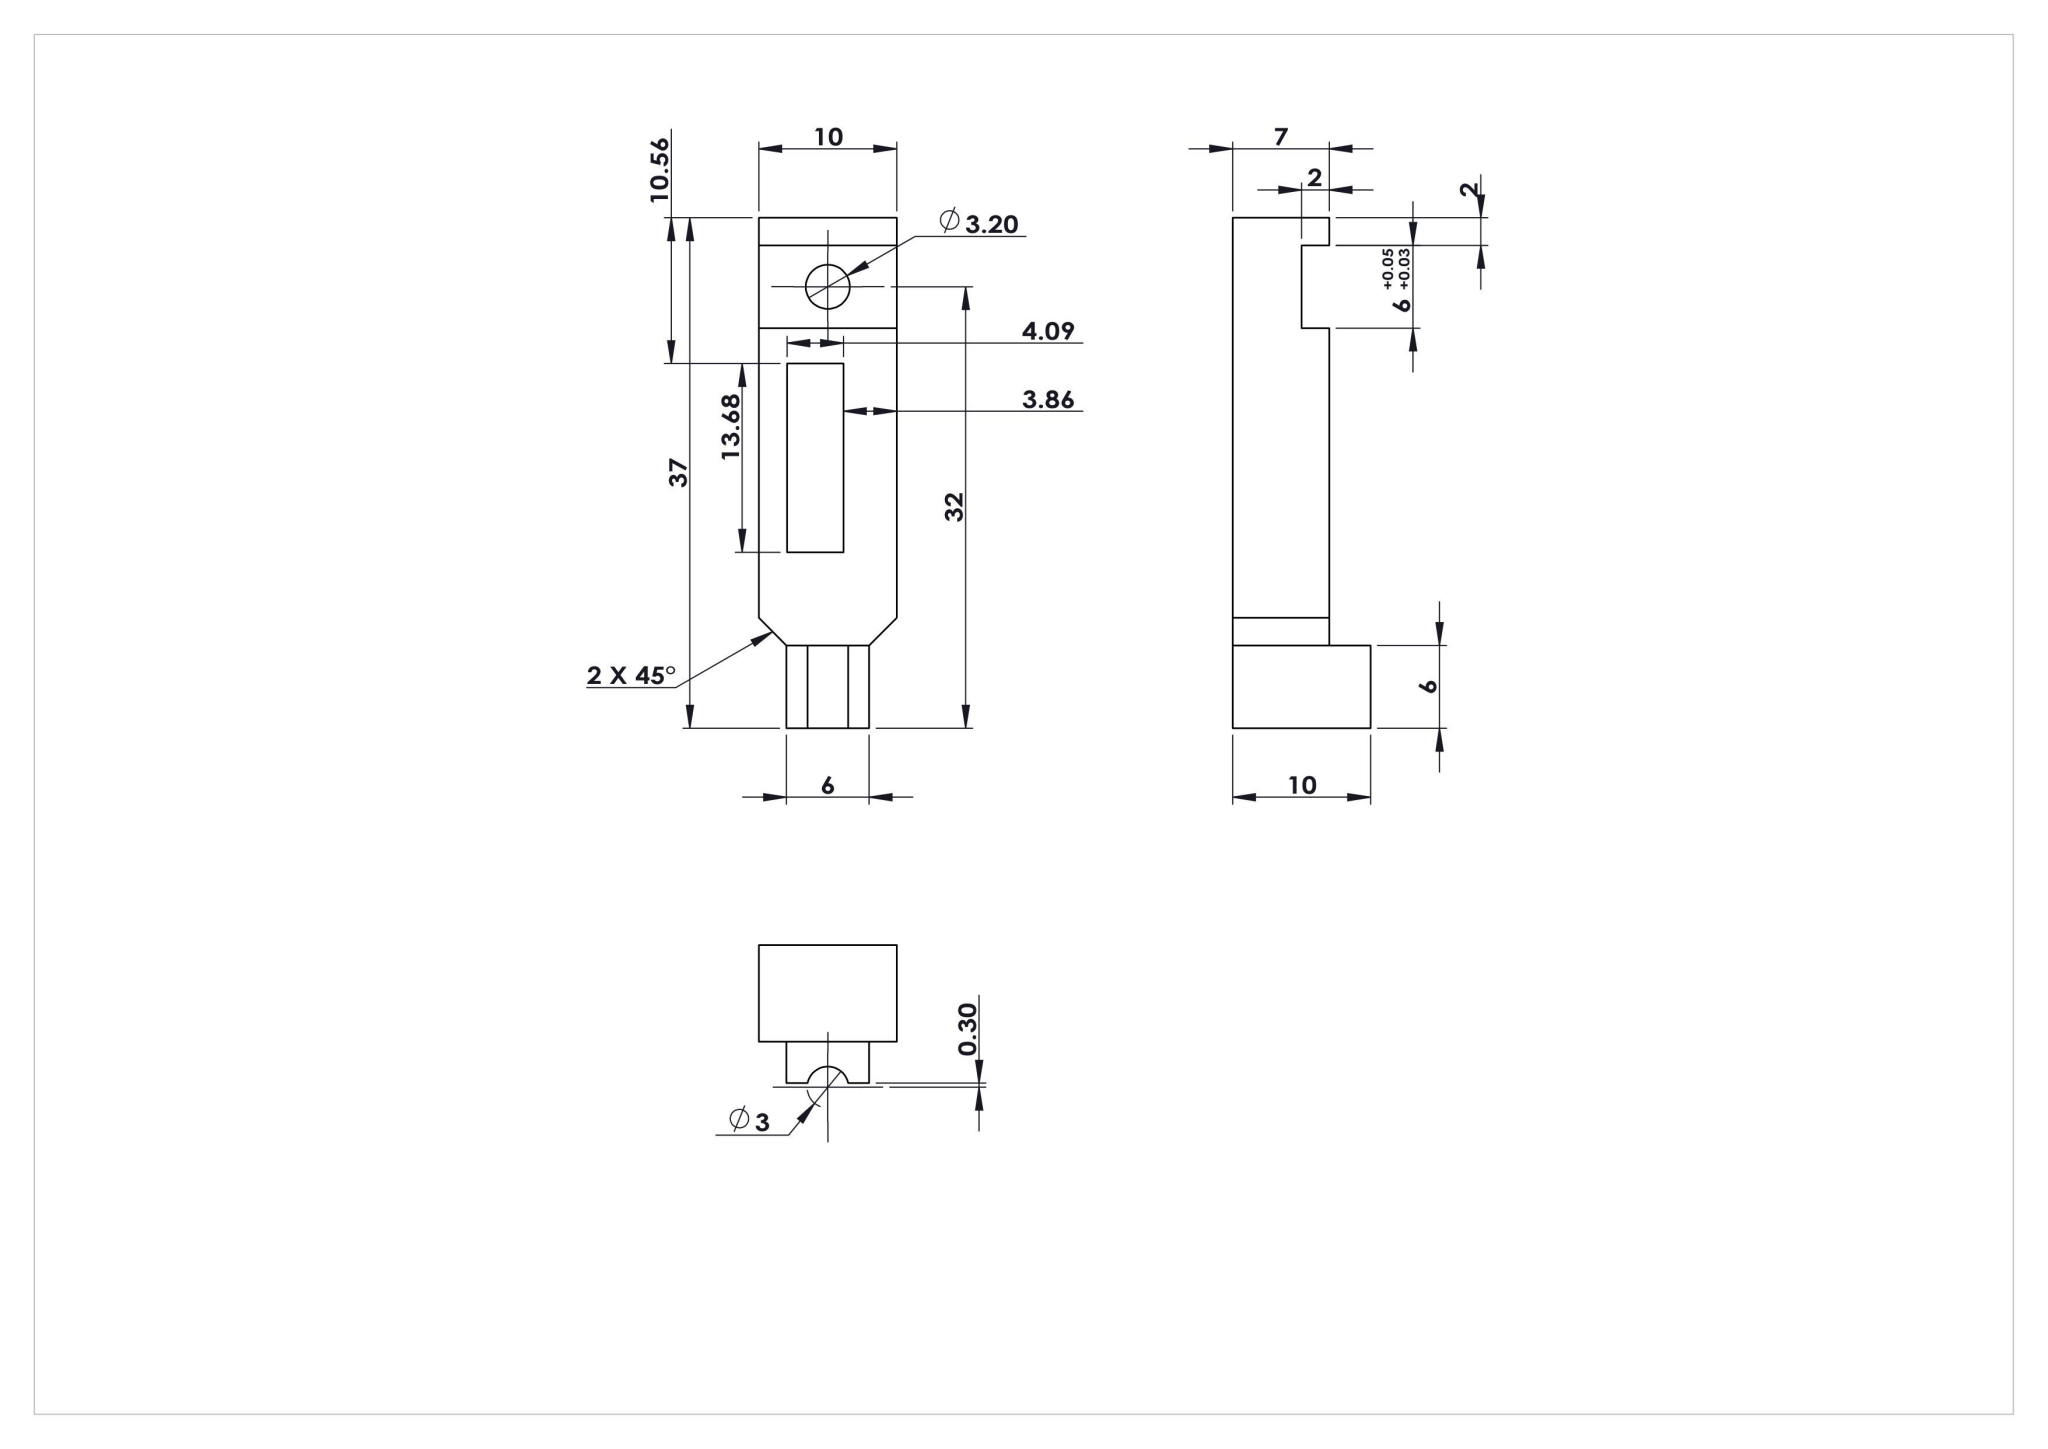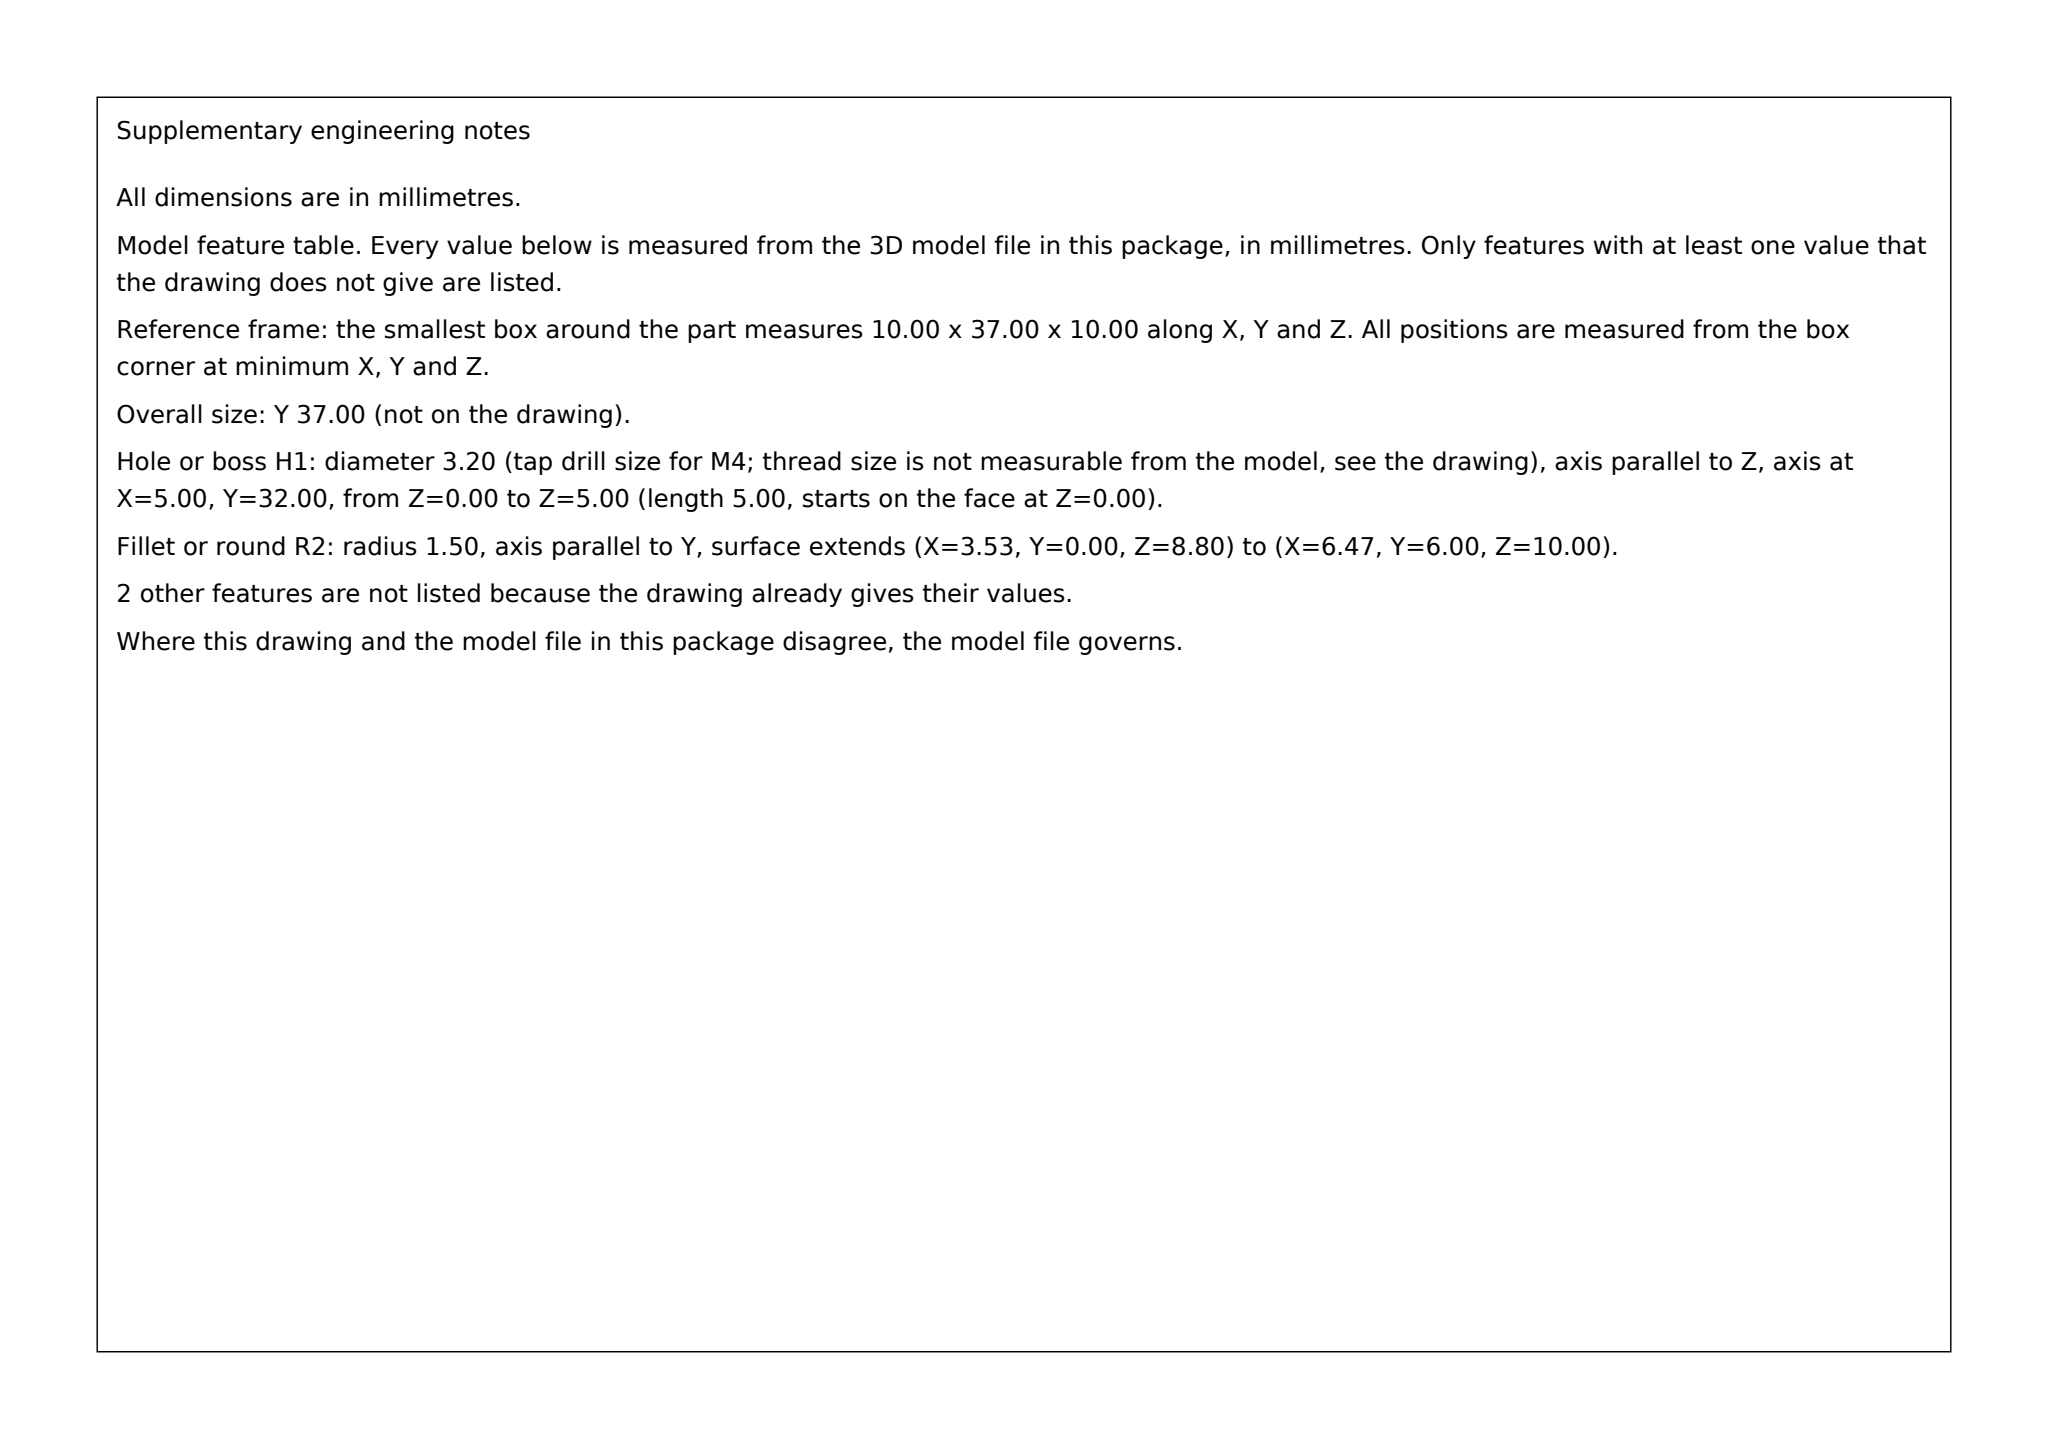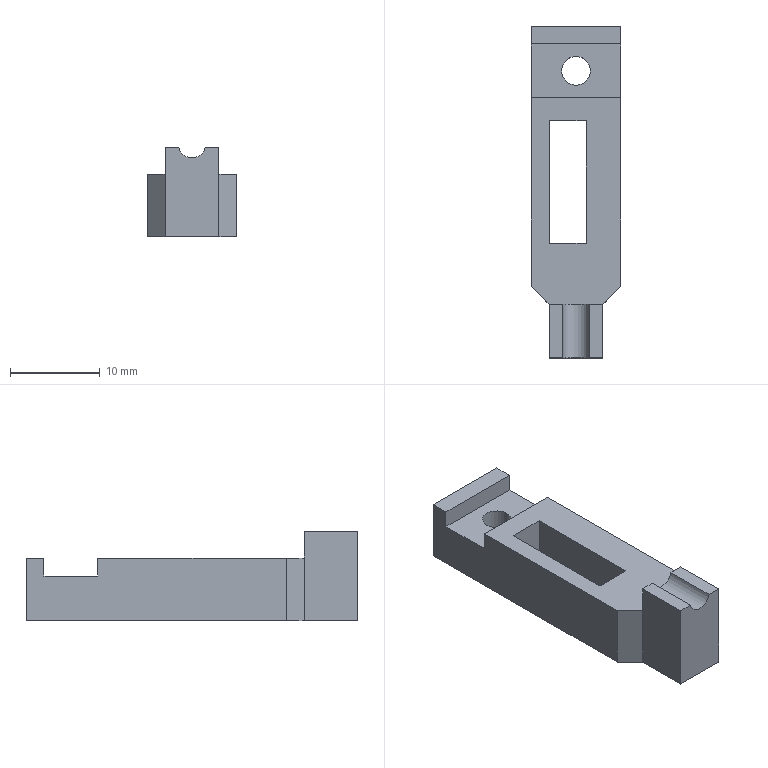Part | SolidWorks | mm | 1 solid | 24 faces | box 10 x 37 x 10 mm | volume 1934 mm3 | plane 21 | cylinder 3 | commonest cylinder face diameters 3.2 x2 3 x1
build123d program:
from build123d import *

# Parameters (mm, degrees)
SKETCH1_W            = 10
SKETCH1_H            = 37
BOSS_EXTRUDE1_DEPTH  = 10
SKETCH2_R            = 1.5
CUT_EXTRUDE1_DEPTH   = 39.652
SKETCH3_W            = 3
SKETCH3_H            = 31
CUT_EXTRUDE2_DEPTH   = 24.286
SKETCH5_W            = 2
SKETCH5_H            = 6
CUT_EXTRUDE4_DEPTH   = 22.616
CUT_EXTRUDE5_DEPTH   = 21.402
SKETCH7_W            = 10
SKETCH7_H            = 6
CUT_EXTRUDE6_DEPTH   = 2
SKETCH1_2_R          = 1.6
CUT_EXTRUDE1_2_DEPTH = 20.805
SKETCH2_2_W          = 4.092
SKETCH2_2_H          = 13.678
CUT_EXTRUDE2_2_DEPTH = 10


with BuildPart() as part:
    # Sketch1 → Boss-Extrude1 (new body)
    with BuildSketch(Plane.XY):
        Rectangle(SKETCH1_W, SKETCH1_H)
    extrude(amount=-BOSS_EXTRUDE1_DEPTH)

    # Sketch2 → Cut-Extrude1 (cut, through all)
    with BuildSketch(Plane(origin=(0, 18.5, 0), x_dir=(1, 0, 0), z_dir=(0, 1, 0))):
        with Locations((0, -0.3)):
            Circle(SKETCH2_R)
    extrude(amount=-CUT_EXTRUDE1_DEPTH, mode=Mode.SUBTRACT)

    # Sketch3 → Cut-Extrude2 (cut, through all)
    with BuildSketch(Plane(origin=(5, 0, 0), x_dir=(0, 0, -1), z_dir=(1, 0, 0))):
        with Locations((1.5, 3)):
            Rectangle(SKETCH3_W, SKETCH3_H)
    extrude(amount=-CUT_EXTRUDE2_DEPTH, mode=Mode.SUBTRACT)

    # Sketch5 → Cut-Extrude4 (cut, through all)
    with BuildSketch(Plane.XY):
        with Locations((-4, -15.5)):
            Rectangle(SKETCH5_W, SKETCH5_H)
        with Locations((4, -15.5)):
            Rectangle(SKETCH5_W, SKETCH5_H)
    extrude(amount=-CUT_EXTRUDE4_DEPTH, mode=Mode.SUBTRACT)

    # Sketch6 → Cut-Extrude5 (cut, through all)
    with BuildSketch(Plane.XY.offset(-3)):
        Polygon((-3, -12.5), (-5, -10.5), (-5, -12.5), align=None)
        Polygon((5, -12.5), (3, -12.5), (5, -10.5), align=None)
    extrude(amount=-CUT_EXTRUDE5_DEPTH, mode=Mode.SUBTRACT)

    # Sketch7 → Cut-Extrude6 (cut)
    with BuildSketch(Plane.XY.offset(-3)):
        with Locations((0, 13.5)):
            Rectangle(SKETCH7_W, SKETCH7_H)
    extrude(amount=-CUT_EXTRUDE6_DEPTH, mode=Mode.SUBTRACT)

    # Sketch1_2 → Cut-Extrude1_2 (cut, through all)
    with BuildSketch(Plane.XY.offset(-5)):
        with Locations((0, 13.5)):
            Circle(SKETCH1_2_R)
    extrude(amount=-CUT_EXTRUDE1_2_DEPTH, mode=Mode.SUBTRACT)

    # Sketch2_2 → Cut-Extrude2_2 (cut)
    with BuildSketch(Plane.XY.offset(-3)):
        with Locations((-0.9093, 1.099)):
            Rectangle(SKETCH2_2_W, SKETCH2_2_H)
    extrude(amount=-CUT_EXTRUDE2_2_DEPTH, mode=Mode.SUBTRACT)


solid = part.part
STEP:
#1=CARTESIAN_POINT('',(-1.6,13.5,-10.));
#2=VERTEX_POINT('',#1);
#3=CARTESIAN_POINT('',(1.6,13.5,-10.));
#4=VERTEX_POINT('',#3);
#5=CARTESIAN_POINT('',(0.,13.5,-10.));
#6=DIRECTION('',(0.,0.,1.));
#7=DIRECTION('',(1.,0.,0.));
#8=AXIS2_PLACEMENT_3D('',#5,#6,#7);
#9=CIRCLE('',#8,1.6);
#10=EDGE_CURVE('',#2,#4,#9,.T.);
#11=ORIENTED_EDGE('',*,*,#10,.F.);
#12=CARTESIAN_POINT('',(-1.6,13.5,-5.));
#13=VERTEX_POINT('',#12);
#14=CARTESIAN_POINT('',(-1.6,13.5,-10.));
#15=DIRECTION('',(0.,0.,1.));
#16=VECTOR('',#15,1000.);
#17=LINE('',#14,#16);
#18=EDGE_CURVE('',#2,#13,#17,.T.);
#19=ORIENTED_EDGE('',*,*,#18,.T.);
#20=CARTESIAN_POINT('',(1.6,13.5,-5.));
#21=VERTEX_POINT('',#20);
#22=CARTESIAN_POINT('',(0.,13.5,-5.));
#23=DIRECTION('',(0.,0.,1.));
#24=DIRECTION('',(1.,0.,0.));
#25=AXIS2_PLACEMENT_3D('',#22,#23,#24);
#26=CIRCLE('',#25,1.6);
#27=EDGE_CURVE('',#13,#21,#26,.T.);
#28=ORIENTED_EDGE('',*,*,#27,.T.);
#29=CARTESIAN_POINT('',(1.6,13.5,-10.));
#30=DIRECTION('',(0.,0.,1.));
#31=VECTOR('',#30,1000.);
#32=LINE('',#29,#31);
#33=EDGE_CURVE('',#4,#21,#32,.T.);
#34=ORIENTED_EDGE('',*,*,#33,.F.);
#35=EDGE_LOOP('',(#11,#19,#28,#34));
#36=FACE_OUTER_BOUND('',#35,.T.);
#37=CARTESIAN_POINT('',(0.,13.5,-10.));
#38=DIRECTION('',(0.,0.,1.));
#39=DIRECTION('',(1.,0.,0.));
#40=AXIS2_PLACEMENT_3D('',#37,#38,#39);
#41=CYLINDRICAL_SURFACE('',#40,1.6);
#42=ADVANCED_FACE('',(#36),#41,.F.);
#43=CARTESIAN_POINT('',(-5.,16.5,-3.));
#44=VERTEX_POINT('',#43);
#45=CARTESIAN_POINT('',(-5.,18.5,-3.));
#46=VERTEX_POINT('',#45);
#47=CARTESIAN_POINT('',(-5.,18.5,-3.));
#48=DIRECTION('',(0.,1.,0.));
#49=VECTOR('',#48,1000.);
#50=LINE('',#47,#49);
#51=EDGE_CURVE('',#44,#46,#50,.T.);
#52=ORIENTED_EDGE('',*,*,#51,.F.);
#53=CARTESIAN_POINT('',(5.,16.5,-3.));
#54=VERTEX_POINT('',#53);
#55=CARTESIAN_POINT('',(-5.,16.5,-3.));
#56=DIRECTION('',(-1.,0.,0.));
#57=VECTOR('',#56,1000.);
#58=LINE('',#55,#57);
#59=EDGE_CURVE('',#54,#44,#58,.T.);
#60=ORIENTED_EDGE('',*,*,#59,.F.);
#61=CARTESIAN_POINT('',(5.,18.5,-3.));
#62=VERTEX_POINT('',#61);
#63=CARTESIAN_POINT('',(5.,18.5,-3.));
#64=DIRECTION('',(0.,1.,0.));
#65=VECTOR('',#64,1000.);
#66=LINE('',#63,#65);
#67=EDGE_CURVE('',#54,#62,#66,.T.);
#68=ORIENTED_EDGE('',*,*,#67,.T.);
#69=CARTESIAN_POINT('',(-5.,18.5,-3.));
#70=DIRECTION('',(1.,0.,0.));
#71=VECTOR('',#70,1000.);
#72=LINE('',#69,#71);
#73=EDGE_CURVE('',#46,#62,#72,.T.);
#74=ORIENTED_EDGE('',*,*,#73,.F.);
#75=EDGE_LOOP('',(#52,#60,#68,#74));
#76=FACE_OUTER_BOUND('',#75,.T.);
#77=CARTESIAN_POINT('',(-5.,18.5,-3.));
#78=DIRECTION('',(0.,0.,-1.));
#79=DIRECTION('',(0.,1.,0.));
#80=AXIS2_PLACEMENT_3D('',#77,#78,#79);
#81=PLANE('',#80);
#82=ADVANCED_FACE('',(#76),#81,.F.);
#83=CARTESIAN_POINT('',(3.,-12.5,0.));
#84=VERTEX_POINT('',#83);
#85=CARTESIAN_POINT('',(3.,-18.5,0.));
#86=VERTEX_POINT('',#85);
#87=CARTESIAN_POINT('',(3.,-18.5,0.));
#88=DIRECTION('',(0.,-1.,0.));
#89=VECTOR('',#88,1000.);
#90=LINE('',#87,#89);
#91=EDGE_CURVE('',#84,#86,#90,.T.);
#92=ORIENTED_EDGE('',*,*,#91,.F.);
#93=CARTESIAN_POINT('',(1.47,-12.5,-0.));
#94=VERTEX_POINT('',#93);
#95=CARTESIAN_POINT('',(-5.,-12.5,-0.));
#96=DIRECTION('',(1.,0.,0.));
#97=VECTOR('',#96,1000.);
#98=LINE('',#95,#97);
#99=EDGE_CURVE('',#94,#84,#98,.T.);
#100=ORIENTED_EDGE('',*,*,#99,.F.);
#101=CARTESIAN_POINT('',(1.47,-18.5,0.));
#102=VERTEX_POINT('',#101);
#103=CARTESIAN_POINT('',(1.47,-18.5,0.));
#104=DIRECTION('',(0.,1.,0.));
#105=VECTOR('',#104,1000.);
#106=LINE('',#103,#105);
#107=EDGE_CURVE('',#102,#94,#106,.T.);
#108=ORIENTED_EDGE('',*,*,#107,.F.);
#109=CARTESIAN_POINT('',(5.,-18.5,0.));
#110=DIRECTION('',(1.,0.,0.));
#111=VECTOR('',#110,1000.);
#112=LINE('',#109,#111);
#113=EDGE_CURVE('',#102,#86,#112,.T.);
#114=ORIENTED_EDGE('',*,*,#113,.T.);
#115=EDGE_LOOP('',(#92,#100,#108,#114));
#116=FACE_OUTER_BOUND('',#115,.T.);
#117=CARTESIAN_POINT('',(0.,0.,0.));
#118=DIRECTION('',(0.,0.,1.));
#119=DIRECTION('',(1.,0.,0.));
#120=AXIS2_PLACEMENT_3D('',#117,#118,#119);
#121=PLANE('',#120);
#122=ADVANCED_FACE('',(#116),#121,.T.);
#123=CARTESIAN_POINT('',(-5.,16.5,-5.));
#124=VERTEX_POINT('',#123);
#125=CARTESIAN_POINT('',(-5.,16.5,-5.));
#126=DIRECTION('',(0.,0.,1.));
#127=VECTOR('',#126,1000.);
#128=LINE('',#125,#127);
#129=EDGE_CURVE('',#124,#44,#128,.T.);
#130=ORIENTED_EDGE('',*,*,#129,.T.);
#131=ORIENTED_EDGE('',*,*,#51,.T.);
#132=CARTESIAN_POINT('',(-5.,18.5,-10.));
#133=VERTEX_POINT('',#132);
#134=CARTESIAN_POINT('',(-5.,18.5,-10.));
#135=DIRECTION('',(0.,0.,1.));
#136=VECTOR('',#135,1000.);
#137=LINE('',#134,#136);
#138=EDGE_CURVE('',#133,#46,#137,.T.);
#139=ORIENTED_EDGE('',*,*,#138,.F.);
#140=CARTESIAN_POINT('',(-5.,-10.5,-10.));
#141=VERTEX_POINT('',#140);
#142=CARTESIAN_POINT('',(-5.,-18.5,-10.));
#143=DIRECTION('',(0.,-1.,0.));
#144=VECTOR('',#143,1000.);
#145=LINE('',#142,#144);
#146=EDGE_CURVE('',#133,#141,#145,.T.);
#147=ORIENTED_EDGE('',*,*,#146,.T.);
#148=CARTESIAN_POINT('',(-5.,-10.5,-3.));
#149=VERTEX_POINT('',#148);
#150=CARTESIAN_POINT('',(-5.,-10.5,-10.));
#151=DIRECTION('',(0.,0.,1.));
#152=VECTOR('',#151,1000.);
#153=LINE('',#150,#152);
#154=EDGE_CURVE('',#141,#149,#153,.T.);
#155=ORIENTED_EDGE('',*,*,#154,.T.);
#156=CARTESIAN_POINT('',(-5.,10.5,-3.));
#157=VERTEX_POINT('',#156);
#158=CARTESIAN_POINT('',(-5.,18.5,-3.));
#159=DIRECTION('',(0.,1.,0.));
#160=VECTOR('',#159,1000.);
#161=LINE('',#158,#160);
#162=EDGE_CURVE('',#149,#157,#161,.T.);
#163=ORIENTED_EDGE('',*,*,#162,.T.);
#164=CARTESIAN_POINT('',(-5.,10.5,-5.));
#165=VERTEX_POINT('',#164);
#166=CARTESIAN_POINT('',(-5.,10.5,-5.));
#167=DIRECTION('',(0.,0.,1.));
#168=VECTOR('',#167,1000.);
#169=LINE('',#166,#168);
#170=EDGE_CURVE('',#165,#157,#169,.T.);
#171=ORIENTED_EDGE('',*,*,#170,.F.);
#172=CARTESIAN_POINT('',(-5.,16.5,-5.));
#173=DIRECTION('',(0.,-1.,0.));
#174=VECTOR('',#173,1000.);
#175=LINE('',#172,#174);
#176=EDGE_CURVE('',#124,#165,#175,.T.);
#177=ORIENTED_EDGE('',*,*,#176,.F.);
#178=EDGE_LOOP('',(#130,#131,#139,#147,#155,#163,#171,#177));
#179=FACE_OUTER_BOUND('',#178,.T.);
#180=CARTESIAN_POINT('',(-5.,-18.5,-10.));
#181=DIRECTION('',(-1.,0.,0.));
#182=DIRECTION('',(0.,0.,1.));
#183=AXIS2_PLACEMENT_3D('',#180,#181,#182);
#184=PLANE('',#183);
#185=ADVANCED_FACE('',(#179),#184,.T.);
#186=ORIENTED_EDGE('',*,*,#73,.T.);
#187=CARTESIAN_POINT('',(5.,18.5,-10.));
#188=VERTEX_POINT('',#187);
#189=CARTESIAN_POINT('',(5.,18.5,-10.));
#190=DIRECTION('',(0.,0.,1.));
#191=VECTOR('',#190,1000.);
#192=LINE('',#189,#191);
#193=EDGE_CURVE('',#188,#62,#192,.T.);
#194=ORIENTED_EDGE('',*,*,#193,.F.);
#195=CARTESIAN_POINT('',(5.,18.5,-10.));
#196=DIRECTION('',(-1.,0.,0.));
#197=VECTOR('',#196,1000.);
#198=LINE('',#195,#197);
#199=EDGE_CURVE('',#188,#133,#198,.T.);
#200=ORIENTED_EDGE('',*,*,#199,.T.);
#201=ORIENTED_EDGE('',*,*,#138,.T.);
#202=EDGE_LOOP('',(#186,#194,#200,#201));
#203=FACE_OUTER_BOUND('',#202,.T.);
#204=CARTESIAN_POINT('',(5.,18.5,-10.));
#205=DIRECTION('',(0.,1.,0.));
#206=DIRECTION('',(0.,0.,1.));
#207=AXIS2_PLACEMENT_3D('',#204,#205,#206);
#208=PLANE('',#207);
#209=ADVANCED_FACE('',(#203),#208,.T.);
#210=CARTESIAN_POINT('',(5.,16.5,-5.));
#211=VERTEX_POINT('',#210);
#212=CARTESIAN_POINT('',(5.,16.5,-5.));
#213=DIRECTION('',(0.,0.,1.));
#214=VECTOR('',#213,1000.);
#215=LINE('',#212,#214);
#216=EDGE_CURVE('',#211,#54,#215,.T.);
#217=ORIENTED_EDGE('',*,*,#216,.F.);
#218=CARTESIAN_POINT('',(5.,10.5,-5.));
#219=VERTEX_POINT('',#218);
#220=CARTESIAN_POINT('',(5.,16.5,-5.));
#221=DIRECTION('',(-0.,1.,0.));
#222=VECTOR('',#221,1000.);
#223=LINE('',#220,#222);
#224=EDGE_CURVE('',#219,#211,#223,.T.);
#225=ORIENTED_EDGE('',*,*,#224,.F.);
#226=CARTESIAN_POINT('',(5.,10.5,-3.));
#227=VERTEX_POINT('',#226);
#228=CARTESIAN_POINT('',(5.,10.5,-5.));
#229=DIRECTION('',(0.,0.,1.));
#230=VECTOR('',#229,1000.);
#231=LINE('',#228,#230);
#232=EDGE_CURVE('',#219,#227,#231,.T.);
#233=ORIENTED_EDGE('',*,*,#232,.T.);
#234=CARTESIAN_POINT('',(5.,-10.5,-3.));
#235=VERTEX_POINT('',#234);
#236=CARTESIAN_POINT('',(5.,18.5,-3.));
#237=DIRECTION('',(0.,1.,0.));
#238=VECTOR('',#237,1000.);
#239=LINE('',#236,#238);
#240=EDGE_CURVE('',#235,#227,#239,.T.);
#241=ORIENTED_EDGE('',*,*,#240,.F.);
#242=CARTESIAN_POINT('',(5.,-10.5,-10.));
#243=VERTEX_POINT('',#242);
#244=CARTESIAN_POINT('',(5.,-10.5,-10.));
#245=DIRECTION('',(0.,0.,1.));
#246=VECTOR('',#245,1000.);
#247=LINE('',#244,#246);
#248=EDGE_CURVE('',#243,#235,#247,.T.);
#249=ORIENTED_EDGE('',*,*,#248,.F.);
#250=CARTESIAN_POINT('',(5.,-18.5,-10.));
#251=DIRECTION('',(0.,1.,0.));
#252=VECTOR('',#251,1000.);
#253=LINE('',#250,#252);
#254=EDGE_CURVE('',#243,#188,#253,.T.);
#255=ORIENTED_EDGE('',*,*,#254,.T.);
#256=ORIENTED_EDGE('',*,*,#193,.T.);
#257=ORIENTED_EDGE('',*,*,#67,.F.);
#258=EDGE_LOOP('',(#217,#225,#233,#241,#249,#255,#256,#257));
#259=FACE_OUTER_BOUND('',#258,.T.);
#260=CARTESIAN_POINT('',(5.,-18.5,-10.));
#261=DIRECTION('',(1.,0.,0.));
#262=DIRECTION('',(0.,0.,-1.));
#263=AXIS2_PLACEMENT_3D('',#260,#261,#262);
#264=PLANE('',#263);
#265=ADVANCED_FACE('',(#259),#264,.T.);
#266=CARTESIAN_POINT('',(3.,-18.5,-10.));
#267=VERTEX_POINT('',#266);
#268=CARTESIAN_POINT('',(3.,-18.5,-10.));
#269=DIRECTION('',(0.,0.,1.));
#270=VECTOR('',#269,1000.);
#271=LINE('',#268,#270);
#272=EDGE_CURVE('',#267,#86,#271,.T.);
#273=ORIENTED_EDGE('',*,*,#272,.T.);
#274=ORIENTED_EDGE('',*,*,#113,.F.);
#275=CARTESIAN_POINT('',(-1.47,-18.5,0.));
#276=VERTEX_POINT('',#275);
#277=CARTESIAN_POINT('',(0.,-18.5,0.3));
#278=DIRECTION('',(0.,1.,0.));
#279=DIRECTION('',(0.,0.,1.));
#280=AXIS2_PLACEMENT_3D('',#277,#278,#279);
#281=CIRCLE('',#280,1.5);
#282=EDGE_CURVE('',#102,#276,#281,.T.);
#283=ORIENTED_EDGE('',*,*,#282,.T.);
#284=CARTESIAN_POINT('',(-3.,-18.5,0.));
#285=VERTEX_POINT('',#284);
#286=CARTESIAN_POINT('',(5.,-18.5,0.));
#287=DIRECTION('',(1.,0.,0.));
#288=VECTOR('',#287,1000.);
#289=LINE('',#286,#288);
#290=EDGE_CURVE('',#285,#276,#289,.T.);
#291=ORIENTED_EDGE('',*,*,#290,.F.);
#292=CARTESIAN_POINT('',(-3.,-18.5,-10.));
#293=VERTEX_POINT('',#292);
#294=CARTESIAN_POINT('',(-3.,-18.5,-10.));
#295=DIRECTION('',(0.,0.,1.));
#296=VECTOR('',#295,1000.);
#297=LINE('',#294,#296);
#298=EDGE_CURVE('',#293,#285,#297,.T.);
#299=ORIENTED_EDGE('',*,*,#298,.F.);
#300=CARTESIAN_POINT('',(5.,-18.5,-10.));
#301=DIRECTION('',(1.,0.,0.));
#302=VECTOR('',#301,1000.);
#303=LINE('',#300,#302);
#304=EDGE_CURVE('',#293,#267,#303,.T.);
#305=ORIENTED_EDGE('',*,*,#304,.T.);
#306=EDGE_LOOP('',(#273,#274,#283,#291,#299,#305));
#307=FACE_OUTER_BOUND('',#306,.T.);
#308=CARTESIAN_POINT('',(5.,-18.5,-10.));
#309=DIRECTION('',(0.,-1.,0.));
#310=DIRECTION('',(0.,0.,-1.));
#311=AXIS2_PLACEMENT_3D('',#308,#309,#310);
#312=PLANE('',#311);
#313=ADVANCED_FACE('',(#307),#312,.T.);
#314=CARTESIAN_POINT('',(1.137,7.938,-10.));
#315=VERTEX_POINT('',#314);
#316=CARTESIAN_POINT('',(-2.955,7.938,-10.));
#317=VERTEX_POINT('',#316);
#318=CARTESIAN_POINT('',(0.,7.938,-10.));
#319=DIRECTION('',(-1.,0.,0.));
#320=VECTOR('',#319,1000.);
#321=LINE('',#318,#320);
#322=EDGE_CURVE('',#315,#317,#321,.T.);
#323=ORIENTED_EDGE('',*,*,#322,.T.);
#324=CARTESIAN_POINT('',(-2.955,-5.74,-10.));
#325=VERTEX_POINT('',#324);
#326=CARTESIAN_POINT('',(-2.955,0.,-10.));
#327=DIRECTION('',(0.,-1.,0.));
#328=VECTOR('',#327,1000.);
#329=LINE('',#326,#328);
#330=EDGE_CURVE('',#317,#325,#329,.T.);
#331=ORIENTED_EDGE('',*,*,#330,.T.);
#332=CARTESIAN_POINT('',(1.137,-5.74,-10.));
#333=VERTEX_POINT('',#332);
#334=CARTESIAN_POINT('',(0.,-5.74,-10.));
#335=DIRECTION('',(1.,0.,0.));
#336=VECTOR('',#335,1000.);
#337=LINE('',#334,#336);
#338=EDGE_CURVE('',#325,#333,#337,.T.);
#339=ORIENTED_EDGE('',*,*,#338,.T.);
#340=CARTESIAN_POINT('',(1.137,0.,-10.));
#341=DIRECTION('',(0.,1.,0.));
#342=VECTOR('',#341,1000.);
#343=LINE('',#340,#342);
#344=EDGE_CURVE('',#333,#315,#343,.T.);
#345=ORIENTED_EDGE('',*,*,#344,.T.);
#346=EDGE_LOOP('',(#323,#331,#339,#345));
#347=FACE_BOUND('',#346,.T.);
#348=CARTESIAN_POINT('',(0.,13.5,-10.));
#349=DIRECTION('',(0.,0.,1.));
#350=DIRECTION('',(1.,0.,0.));
#351=AXIS2_PLACEMENT_3D('',#348,#349,#350);
#352=CIRCLE('',#351,1.6);
#353=EDGE_CURVE('',#4,#2,#352,.T.);
#354=ORIENTED_EDGE('',*,*,#353,.T.);
#355=ORIENTED_EDGE('',*,*,#10,.T.);
#356=EDGE_LOOP('',(#354,#355));
#357=FACE_BOUND('',#356,.T.);
#358=ORIENTED_EDGE('',*,*,#254,.F.);
#359=CARTESIAN_POINT('',(3.,-12.5,-10.));
#360=VERTEX_POINT('',#359);
#361=CARTESIAN_POINT('',(3.,-12.5,-10.));
#362=DIRECTION('',(-0.7071,-0.7071,0.));
#363=VECTOR('',#362,1000.);
#364=LINE('',#361,#363);
#365=EDGE_CURVE('',#243,#360,#364,.T.);
#366=ORIENTED_EDGE('',*,*,#365,.T.);
#367=CARTESIAN_POINT('',(3.,-18.5,-10.));
#368=DIRECTION('',(0.,-1.,0.));
#369=VECTOR('',#368,1000.);
#370=LINE('',#367,#369);
#371=EDGE_CURVE('',#360,#267,#370,.T.);
#372=ORIENTED_EDGE('',*,*,#371,.T.);
#373=ORIENTED_EDGE('',*,*,#304,.F.);
#374=CARTESIAN_POINT('',(-3.,-12.5,-10.));
#375=VERTEX_POINT('',#374);
#376=CARTESIAN_POINT('',(-3.,-18.5,-10.));
#377=DIRECTION('',(0.,1.,0.));
#378=VECTOR('',#377,1000.);
#379=LINE('',#376,#378);
#380=EDGE_CURVE('',#293,#375,#379,.T.);
#381=ORIENTED_EDGE('',*,*,#380,.T.);
#382=CARTESIAN_POINT('',(-3.,-12.5,-10.));
#383=DIRECTION('',(-0.7071,0.7071,0.));
#384=VECTOR('',#383,1000.);
#385=LINE('',#382,#384);
#386=EDGE_CURVE('',#375,#141,#385,.T.);
#387=ORIENTED_EDGE('',*,*,#386,.T.);
#388=ORIENTED_EDGE('',*,*,#146,.F.);
#389=ORIENTED_EDGE('',*,*,#199,.F.);
#390=EDGE_LOOP('',(#358,#366,#372,#373,#381,#387,#388,#389));
#391=FACE_OUTER_BOUND('',#390,.T.);
#392=CARTESIAN_POINT('',(0.,0.,-10.));
#393=DIRECTION('',(0.,0.,1.));
#394=DIRECTION('',(1.,0.,0.));
#395=AXIS2_PLACEMENT_3D('',#392,#393,#394);
#396=PLANE('',#395);
#397=ADVANCED_FACE('',(#347,#357,#391),#396,.F.);
#398=CARTESIAN_POINT('',(-3.,-12.5,0.));
#399=VERTEX_POINT('',#398);
#400=CARTESIAN_POINT('',(-3.,-18.5,0.));
#401=DIRECTION('',(0.,1.,0.));
#402=VECTOR('',#401,1000.);
#403=LINE('',#400,#402);
#404=EDGE_CURVE('',#285,#399,#403,.T.);
#405=ORIENTED_EDGE('',*,*,#404,.F.);
#406=ORIENTED_EDGE('',*,*,#290,.T.);
#407=CARTESIAN_POINT('',(-1.47,-12.5,0.));
#408=VERTEX_POINT('',#407);
#409=CARTESIAN_POINT('',(-1.47,-18.5,0.));
#410=DIRECTION('',(0.,-1.,0.));
#411=VECTOR('',#410,1000.);
#412=LINE('',#409,#411);
#413=EDGE_CURVE('',#408,#276,#412,.T.);
#414=ORIENTED_EDGE('',*,*,#413,.F.);
#415=CARTESIAN_POINT('',(-5.,-12.5,-0.));
#416=DIRECTION('',(1.,0.,0.));
#417=VECTOR('',#416,1000.);
#418=LINE('',#415,#417);
#419=EDGE_CURVE('',#399,#408,#418,.T.);
#420=ORIENTED_EDGE('',*,*,#419,.F.);
#421=EDGE_LOOP('',(#405,#406,#414,#420));
#422=FACE_OUTER_BOUND('',#421,.T.);
#423=CARTESIAN_POINT('',(0.,0.,0.));
#424=DIRECTION('',(0.,0.,1.));
#425=DIRECTION('',(1.,0.,0.));
#426=AXIS2_PLACEMENT_3D('',#423,#424,#425);
#427=PLANE('',#426);
#428=ADVANCED_FACE('',(#422),#427,.T.);
#429=ORIENTED_EDGE('',*,*,#107,.T.);
#430=CARTESIAN_POINT('',(0.,-12.5,0.3));
#431=DIRECTION('',(0.,1.,-0.));
#432=DIRECTION('',(0.,-0.,-1.));
#433=AXIS2_PLACEMENT_3D('',#430,#431,#432);
#434=CIRCLE('',#433,1.5);
#435=EDGE_CURVE('',#94,#408,#434,.T.);
#436=ORIENTED_EDGE('',*,*,#435,.T.);
#437=ORIENTED_EDGE('',*,*,#413,.T.);
#438=ORIENTED_EDGE('',*,*,#282,.F.);
#439=EDGE_LOOP('',(#429,#436,#437,#438));
#440=FACE_OUTER_BOUND('',#439,.T.);
#441=CARTESIAN_POINT('',(0.,-18.5,0.3));
#442=DIRECTION('',(0.,1.,0.));
#443=DIRECTION('',(0.,0.,1.));
#444=AXIS2_PLACEMENT_3D('',#441,#442,#443);
#445=CYLINDRICAL_SURFACE('',#444,1.5);
#446=ADVANCED_FACE('',(#440),#445,.F.);
#447=ORIENTED_EDGE('',*,*,#99,.T.);
#448=CARTESIAN_POINT('',(3.,-12.5,-3.));
#449=VERTEX_POINT('',#448);
#450=CARTESIAN_POINT('',(3.,-12.5,-10.));
#451=DIRECTION('',(0.,0.,1.));
#452=VECTOR('',#451,1000.);
#453=LINE('',#450,#452);
#454=EDGE_CURVE('',#449,#84,#453,.T.);
#455=ORIENTED_EDGE('',*,*,#454,.F.);
#456=CARTESIAN_POINT('',(-3.,-12.5,-3.));
#457=VERTEX_POINT('',#456);
#458=CARTESIAN_POINT('',(-5.,-12.5,-3.));
#459=DIRECTION('',(1.,0.,0.));
#460=VECTOR('',#459,1000.);
#461=LINE('',#458,#460);
#462=EDGE_CURVE('',#457,#449,#461,.T.);
#463=ORIENTED_EDGE('',*,*,#462,.F.);
#464=CARTESIAN_POINT('',(-3.,-12.5,-10.));
#465=DIRECTION('',(0.,0.,1.));
#466=VECTOR('',#465,1000.);
#467=LINE('',#464,#466);
#468=EDGE_CURVE('',#457,#399,#467,.T.);
#469=ORIENTED_EDGE('',*,*,#468,.T.);
#470=ORIENTED_EDGE('',*,*,#419,.T.);
#471=ORIENTED_EDGE('',*,*,#435,.F.);
#472=EDGE_LOOP('',(#447,#455,#463,#469,#470,#471));
#473=FACE_OUTER_BOUND('',#472,.T.);
#474=CARTESIAN_POINT('',(-5.,-12.5,-0.));
#475=DIRECTION('',(0.,-1.,0.));
#476=DIRECTION('',(0.,-0.,-1.));
#477=AXIS2_PLACEMENT_3D('',#474,#475,#476);
#478=PLANE('',#477);
#479=ADVANCED_FACE('',(#473),#478,.F.);
#480=CARTESIAN_POINT('',(-2.955,-5.74,-3.));
#481=VERTEX_POINT('',#480);
#482=CARTESIAN_POINT('',(1.137,-5.74,-3.));
#483=VERTEX_POINT('',#482);
#484=CARTESIAN_POINT('',(-2.955,-5.74,-3.));
#485=DIRECTION('',(1.,0.,0.));
#486=VECTOR('',#485,1000.);
#487=LINE('',#484,#486);
#488=EDGE_CURVE('',#481,#483,#487,.T.);
#489=ORIENTED_EDGE('',*,*,#488,.F.);
#490=CARTESIAN_POINT('',(-2.955,7.938,-3.));
#491=VERTEX_POINT('',#490);
#492=CARTESIAN_POINT('',(-2.955,7.938,-3.));
#493=DIRECTION('',(0.,-1.,0.));
#494=VECTOR('',#493,1000.);
#495=LINE('',#492,#494);
#496=EDGE_CURVE('',#491,#481,#495,.T.);
#497=ORIENTED_EDGE('',*,*,#496,.F.);
#498=CARTESIAN_POINT('',(1.137,7.938,-3.));
#499=VERTEX_POINT('',#498);
#500=CARTESIAN_POINT('',(-2.955,7.938,-3.));
#501=DIRECTION('',(-1.,0.,0.));
#502=VECTOR('',#501,1000.);
#503=LINE('',#500,#502);
#504=EDGE_CURVE('',#499,#491,#503,.T.);
#505=ORIENTED_EDGE('',*,*,#504,.F.);
#506=CARTESIAN_POINT('',(1.137,7.938,-3.));
#507=DIRECTION('',(0.,1.,0.));
#508=VECTOR('',#507,1000.);
#509=LINE('',#506,#508);
#510=EDGE_CURVE('',#483,#499,#509,.T.);
#511=ORIENTED_EDGE('',*,*,#510,.F.);
#512=EDGE_LOOP('',(#489,#497,#505,#511));
#513=FACE_BOUND('',#512,.T.);
#514=ORIENTED_EDGE('',*,*,#240,.T.);
#515=CARTESIAN_POINT('',(-5.,10.5,-3.));
#516=DIRECTION('',(1.,-0.,0.));
#517=VECTOR('',#516,1000.);
#518=LINE('',#515,#517);
#519=EDGE_CURVE('',#157,#227,#518,.T.);
#520=ORIENTED_EDGE('',*,*,#519,.F.);
#521=ORIENTED_EDGE('',*,*,#162,.F.);
#522=CARTESIAN_POINT('',(-3.,-12.5,-3.));
#523=DIRECTION('',(-0.7071,0.7071,0.));
#524=VECTOR('',#523,1000.);
#525=LINE('',#522,#524);
#526=EDGE_CURVE('',#457,#149,#525,.T.);
#527=ORIENTED_EDGE('',*,*,#526,.F.);
#528=ORIENTED_EDGE('',*,*,#462,.T.);
#529=CARTESIAN_POINT('',(3.,-12.5,-3.));
#530=DIRECTION('',(-0.7071,-0.7071,0.));
#531=VECTOR('',#530,1000.);
#532=LINE('',#529,#531);
#533=EDGE_CURVE('',#235,#449,#532,.T.);
#534=ORIENTED_EDGE('',*,*,#533,.F.);
#535=EDGE_LOOP('',(#514,#520,#521,#527,#528,#534));
#536=FACE_OUTER_BOUND('',#535,.T.);
#537=CARTESIAN_POINT('',(-5.,18.5,-3.));
#538=DIRECTION('',(0.,0.,-1.));
#539=DIRECTION('',(0.,1.,0.));
#540=AXIS2_PLACEMENT_3D('',#537,#538,#539);
#541=PLANE('',#540);
#542=ADVANCED_FACE('',(#513,#536),#541,.F.);
#543=ORIENTED_EDGE('',*,*,#404,.T.);
#544=ORIENTED_EDGE('',*,*,#468,.F.);
#545=CARTESIAN_POINT('',(-3.,-12.5,-10.));
#546=DIRECTION('',(0.,0.,1.));
#547=VECTOR('',#546,1000.);
#548=LINE('',#545,#547);
#549=EDGE_CURVE('',#375,#457,#548,.T.);
#550=ORIENTED_EDGE('',*,*,#549,.F.);
#551=ORIENTED_EDGE('',*,*,#380,.F.);
#552=ORIENTED_EDGE('',*,*,#298,.T.);
#553=EDGE_LOOP('',(#543,#544,#550,#551,#552));
#554=FACE_OUTER_BOUND('',#553,.T.);
#555=CARTESIAN_POINT('',(-3.,-18.5,-10.));
#556=DIRECTION('',(1.,0.,0.));
#557=DIRECTION('',(0.,0.,-1.));
#558=AXIS2_PLACEMENT_3D('',#555,#556,#557);
#559=PLANE('',#558);
#560=ADVANCED_FACE('',(#554),#559,.F.);
#561=ORIENTED_EDGE('',*,*,#91,.T.);
#562=ORIENTED_EDGE('',*,*,#272,.F.);
#563=ORIENTED_EDGE('',*,*,#371,.F.);
#564=CARTESIAN_POINT('',(3.,-12.5,-10.));
#565=DIRECTION('',(0.,0.,1.));
#566=VECTOR('',#565,1000.);
#567=LINE('',#564,#566);
#568=EDGE_CURVE('',#360,#449,#567,.T.);
#569=ORIENTED_EDGE('',*,*,#568,.T.);
#570=ORIENTED_EDGE('',*,*,#454,.T.);
#571=EDGE_LOOP('',(#561,#562,#563,#569,#570));
#572=FACE_OUTER_BOUND('',#571,.T.);
#573=CARTESIAN_POINT('',(3.,-18.5,-10.));
#574=DIRECTION('',(-1.,-0.,0.));
#575=DIRECTION('',(0.,-1.,0.));
#576=AXIS2_PLACEMENT_3D('',#573,#574,#575);
#577=PLANE('',#576);
#578=ADVANCED_FACE('',(#572),#577,.F.);
#579=ORIENTED_EDGE('',*,*,#526,.T.);
#580=ORIENTED_EDGE('',*,*,#154,.F.);
#581=ORIENTED_EDGE('',*,*,#386,.F.);
#582=ORIENTED_EDGE('',*,*,#549,.T.);
#583=EDGE_LOOP('',(#579,#580,#581,#582));
#584=FACE_OUTER_BOUND('',#583,.T.);
#585=CARTESIAN_POINT('',(-3.,-12.5,-10.));
#586=DIRECTION('',(0.7071,0.7071,0.));
#587=DIRECTION('',(-0.7071,0.7071,0.));
#588=AXIS2_PLACEMENT_3D('',#585,#586,#587);
#589=PLANE('',#588);
#590=ADVANCED_FACE('',(#584),#589,.F.);
#591=ORIENTED_EDGE('',*,*,#533,.T.);
#592=ORIENTED_EDGE('',*,*,#568,.F.);
#593=ORIENTED_EDGE('',*,*,#365,.F.);
#594=ORIENTED_EDGE('',*,*,#248,.T.);
#595=EDGE_LOOP('',(#591,#592,#593,#594));
#596=FACE_OUTER_BOUND('',#595,.T.);
#597=CARTESIAN_POINT('',(3.,-12.5,-10.));
#598=DIRECTION('',(-0.7071,0.7071,0.));
#599=DIRECTION('',(-0.7071,-0.7071,0.));
#600=AXIS2_PLACEMENT_3D('',#597,#598,#599);
#601=PLANE('',#600);
#602=ADVANCED_FACE('',(#596),#601,.F.);
#603=ORIENTED_EDGE('',*,*,#59,.T.);
#604=ORIENTED_EDGE('',*,*,#129,.F.);
#605=CARTESIAN_POINT('',(-5.,16.5,-5.));
#606=DIRECTION('',(-1.,0.,0.));
#607=VECTOR('',#606,1000.);
#608=LINE('',#605,#607);
#609=EDGE_CURVE('',#211,#124,#608,.T.);
#610=ORIENTED_EDGE('',*,*,#609,.F.);
#611=ORIENTED_EDGE('',*,*,#216,.T.);
#612=EDGE_LOOP('',(#603,#604,#610,#611));
#613=FACE_OUTER_BOUND('',#612,.T.);
#614=CARTESIAN_POINT('',(-5.,16.5,-5.));
#615=DIRECTION('',(0.,1.,0.));
#616=DIRECTION('',(0.,0.,1.));
#617=AXIS2_PLACEMENT_3D('',#614,#615,#616);
#618=PLANE('',#617);
#619=ADVANCED_FACE('',(#613),#618,.F.);
#620=ORIENTED_EDGE('',*,*,#519,.T.);
#621=ORIENTED_EDGE('',*,*,#232,.F.);
#622=CARTESIAN_POINT('',(-5.,10.5,-5.));
#623=DIRECTION('',(1.,-0.,0.));
#624=VECTOR('',#623,1000.);
#625=LINE('',#622,#624);
#626=EDGE_CURVE('',#165,#219,#625,.T.);
#627=ORIENTED_EDGE('',*,*,#626,.F.);
#628=ORIENTED_EDGE('',*,*,#170,.T.);
#629=EDGE_LOOP('',(#620,#621,#627,#628));
#630=FACE_OUTER_BOUND('',#629,.T.);
#631=CARTESIAN_POINT('',(-5.,10.5,-5.));
#632=DIRECTION('',(-0.,-1.,0.));
#633=DIRECTION('',(1.,-0.,0.));
#634=AXIS2_PLACEMENT_3D('',#631,#632,#633);
#635=PLANE('',#634);
#636=ADVANCED_FACE('',(#630),#635,.F.);
#637=CARTESIAN_POINT('',(0.,13.5,-5.));
#638=DIRECTION('',(0.,0.,1.));
#639=DIRECTION('',(1.,0.,0.));
#640=AXIS2_PLACEMENT_3D('',#637,#638,#639);
#641=CIRCLE('',#640,1.6);
#642=EDGE_CURVE('',#21,#13,#641,.T.);
#643=ORIENTED_EDGE('',*,*,#642,.F.);
#644=ORIENTED_EDGE('',*,*,#27,.F.);
#645=EDGE_LOOP('',(#643,#644));
#646=FACE_BOUND('',#645,.T.);
#647=ORIENTED_EDGE('',*,*,#176,.T.);
#648=ORIENTED_EDGE('',*,*,#626,.T.);
#649=ORIENTED_EDGE('',*,*,#224,.T.);
#650=ORIENTED_EDGE('',*,*,#609,.T.);
#651=EDGE_LOOP('',(#647,#648,#649,#650));
#652=FACE_OUTER_BOUND('',#651,.T.);
#653=CARTESIAN_POINT('',(0.,0.,-5.));
#654=DIRECTION('',(0.,0.,1.));
#655=DIRECTION('',(1.,0.,0.));
#656=AXIS2_PLACEMENT_3D('',#653,#654,#655);
#657=PLANE('',#656);
#658=ADVANCED_FACE('',(#646,#652),#657,.T.);
#659=ORIENTED_EDGE('',*,*,#18,.F.);
#660=ORIENTED_EDGE('',*,*,#353,.F.);
#661=ORIENTED_EDGE('',*,*,#33,.T.);
#662=ORIENTED_EDGE('',*,*,#642,.T.);
#663=EDGE_LOOP('',(#659,#660,#661,#662));
#664=FACE_OUTER_BOUND('',#663,.T.);
#665=CARTESIAN_POINT('',(0.,13.5,-10.));
#666=DIRECTION('',(0.,0.,1.));
#667=DIRECTION('',(1.,0.,0.));
#668=AXIS2_PLACEMENT_3D('',#665,#666,#667);
#669=CYLINDRICAL_SURFACE('',#668,1.6);
#670=ADVANCED_FACE('',(#664),#669,.F.);
#671=CARTESIAN_POINT('',(-2.955,7.938,-13.));
#672=DIRECTION('',(0.,0.,1.));
#673=VECTOR('',#672,1000.);
#674=LINE('',#671,#673);
#675=EDGE_CURVE('',#317,#491,#674,.T.);
#676=ORIENTED_EDGE('',*,*,#675,.T.);
#677=ORIENTED_EDGE('',*,*,#496,.T.);
#678=CARTESIAN_POINT('',(-2.955,-5.74,-13.));
#679=DIRECTION('',(0.,0.,1.));
#680=VECTOR('',#679,1000.);
#681=LINE('',#678,#680);
#682=EDGE_CURVE('',#325,#481,#681,.T.);
#683=ORIENTED_EDGE('',*,*,#682,.F.);
#684=ORIENTED_EDGE('',*,*,#330,.F.);
#685=EDGE_LOOP('',(#676,#677,#683,#684));
#686=FACE_OUTER_BOUND('',#685,.T.);
#687=CARTESIAN_POINT('',(-2.955,7.938,-13.));
#688=DIRECTION('',(-1.,0.,0.));
#689=DIRECTION('',(0.,0.,1.));
#690=AXIS2_PLACEMENT_3D('',#687,#688,#689);
#691=PLANE('',#690);
#692=ADVANCED_FACE('',(#686),#691,.F.);
#693=CARTESIAN_POINT('',(1.137,7.938,-13.));
#694=DIRECTION('',(0.,0.,1.));
#695=VECTOR('',#694,1000.);
#696=LINE('',#693,#695);
#697=EDGE_CURVE('',#315,#499,#696,.T.);
#698=ORIENTED_EDGE('',*,*,#697,.T.);
#699=ORIENTED_EDGE('',*,*,#504,.T.);
#700=ORIENTED_EDGE('',*,*,#675,.F.);
#701=ORIENTED_EDGE('',*,*,#322,.F.);
#702=EDGE_LOOP('',(#698,#699,#700,#701));
#703=FACE_OUTER_BOUND('',#702,.T.);
#704=CARTESIAN_POINT('',(-2.955,7.938,-13.));
#705=DIRECTION('',(0.,1.,0.));
#706=DIRECTION('',(0.,0.,1.));
#707=AXIS2_PLACEMENT_3D('',#704,#705,#706);
#708=PLANE('',#707);
#709=ADVANCED_FACE('',(#703),#708,.F.);
#710=CARTESIAN_POINT('',(1.137,-5.74,-13.));
#711=DIRECTION('',(0.,0.,1.));
#712=VECTOR('',#711,1000.);
#713=LINE('',#710,#712);
#714=EDGE_CURVE('',#333,#483,#713,.T.);
#715=ORIENTED_EDGE('',*,*,#714,.T.);
#716=ORIENTED_EDGE('',*,*,#510,.T.);
#717=ORIENTED_EDGE('',*,*,#697,.F.);
#718=ORIENTED_EDGE('',*,*,#344,.F.);
#719=EDGE_LOOP('',(#715,#716,#717,#718));
#720=FACE_OUTER_BOUND('',#719,.T.);
#721=CARTESIAN_POINT('',(1.137,7.938,-13.));
#722=DIRECTION('',(1.,0.,0.));
#723=DIRECTION('',(0.,0.,-1.));
#724=AXIS2_PLACEMENT_3D('',#721,#722,#723);
#725=PLANE('',#724);
#726=ADVANCED_FACE('',(#720),#725,.F.);
#727=ORIENTED_EDGE('',*,*,#682,.T.);
#728=ORIENTED_EDGE('',*,*,#488,.T.);
#729=ORIENTED_EDGE('',*,*,#714,.F.);
#730=ORIENTED_EDGE('',*,*,#338,.F.);
#731=EDGE_LOOP('',(#727,#728,#729,#730));
#732=FACE_OUTER_BOUND('',#731,.T.);
#733=CARTESIAN_POINT('',(-2.955,-5.74,-13.));
#734=DIRECTION('',(0.,-1.,0.));
#735=DIRECTION('',(0.,0.,-1.));
#736=AXIS2_PLACEMENT_3D('',#733,#734,#735);
#737=PLANE('',#736);
#738=ADVANCED_FACE('',(#732),#737,.F.);
#739=CLOSED_SHELL('',(#42,#82,#122,#185,#209,#265,#313,#397,#428,#446,#479,#542,#560,#578,#590,#602,#619,#636,#658,#670,#692,#709,#726,#738));
#740=MANIFOLD_SOLID_BREP('',#739);
#741=CARTESIAN_POINT('',(0.,0.,0.));
#742=DIRECTION('',(0.,0.,1.));
#743=DIRECTION('',(1.,0.,0.));
#744=AXIS2_PLACEMENT_3D('',#741,#742,#743);
#745=(LENGTH_UNIT()NAMED_UNIT(*)SI_UNIT(.MILLI.,.METRE.));
#746=UNCERTAINTY_MEASURE_WITH_UNIT(LENGTH_MEASURE(0.00001),#745,'','');
#747=(NAMED_UNIT(*)PLANE_ANGLE_UNIT()SI_UNIT($,.RADIAN.));
#748=(NAMED_UNIT(*)SI_UNIT($,.STERADIAN.)SOLID_ANGLE_UNIT());
#749=(GEOMETRIC_REPRESENTATION_CONTEXT(3)GLOBAL_UNCERTAINTY_ASSIGNED_CONTEXT((#746))GLOBAL_UNIT_ASSIGNED_CONTEXT((#745,#747,#748))REPRESENTATION_CONTEXT('',''));
#750=ADVANCED_BREP_SHAPE_REPRESENTATION('',(#740,#744),#749);